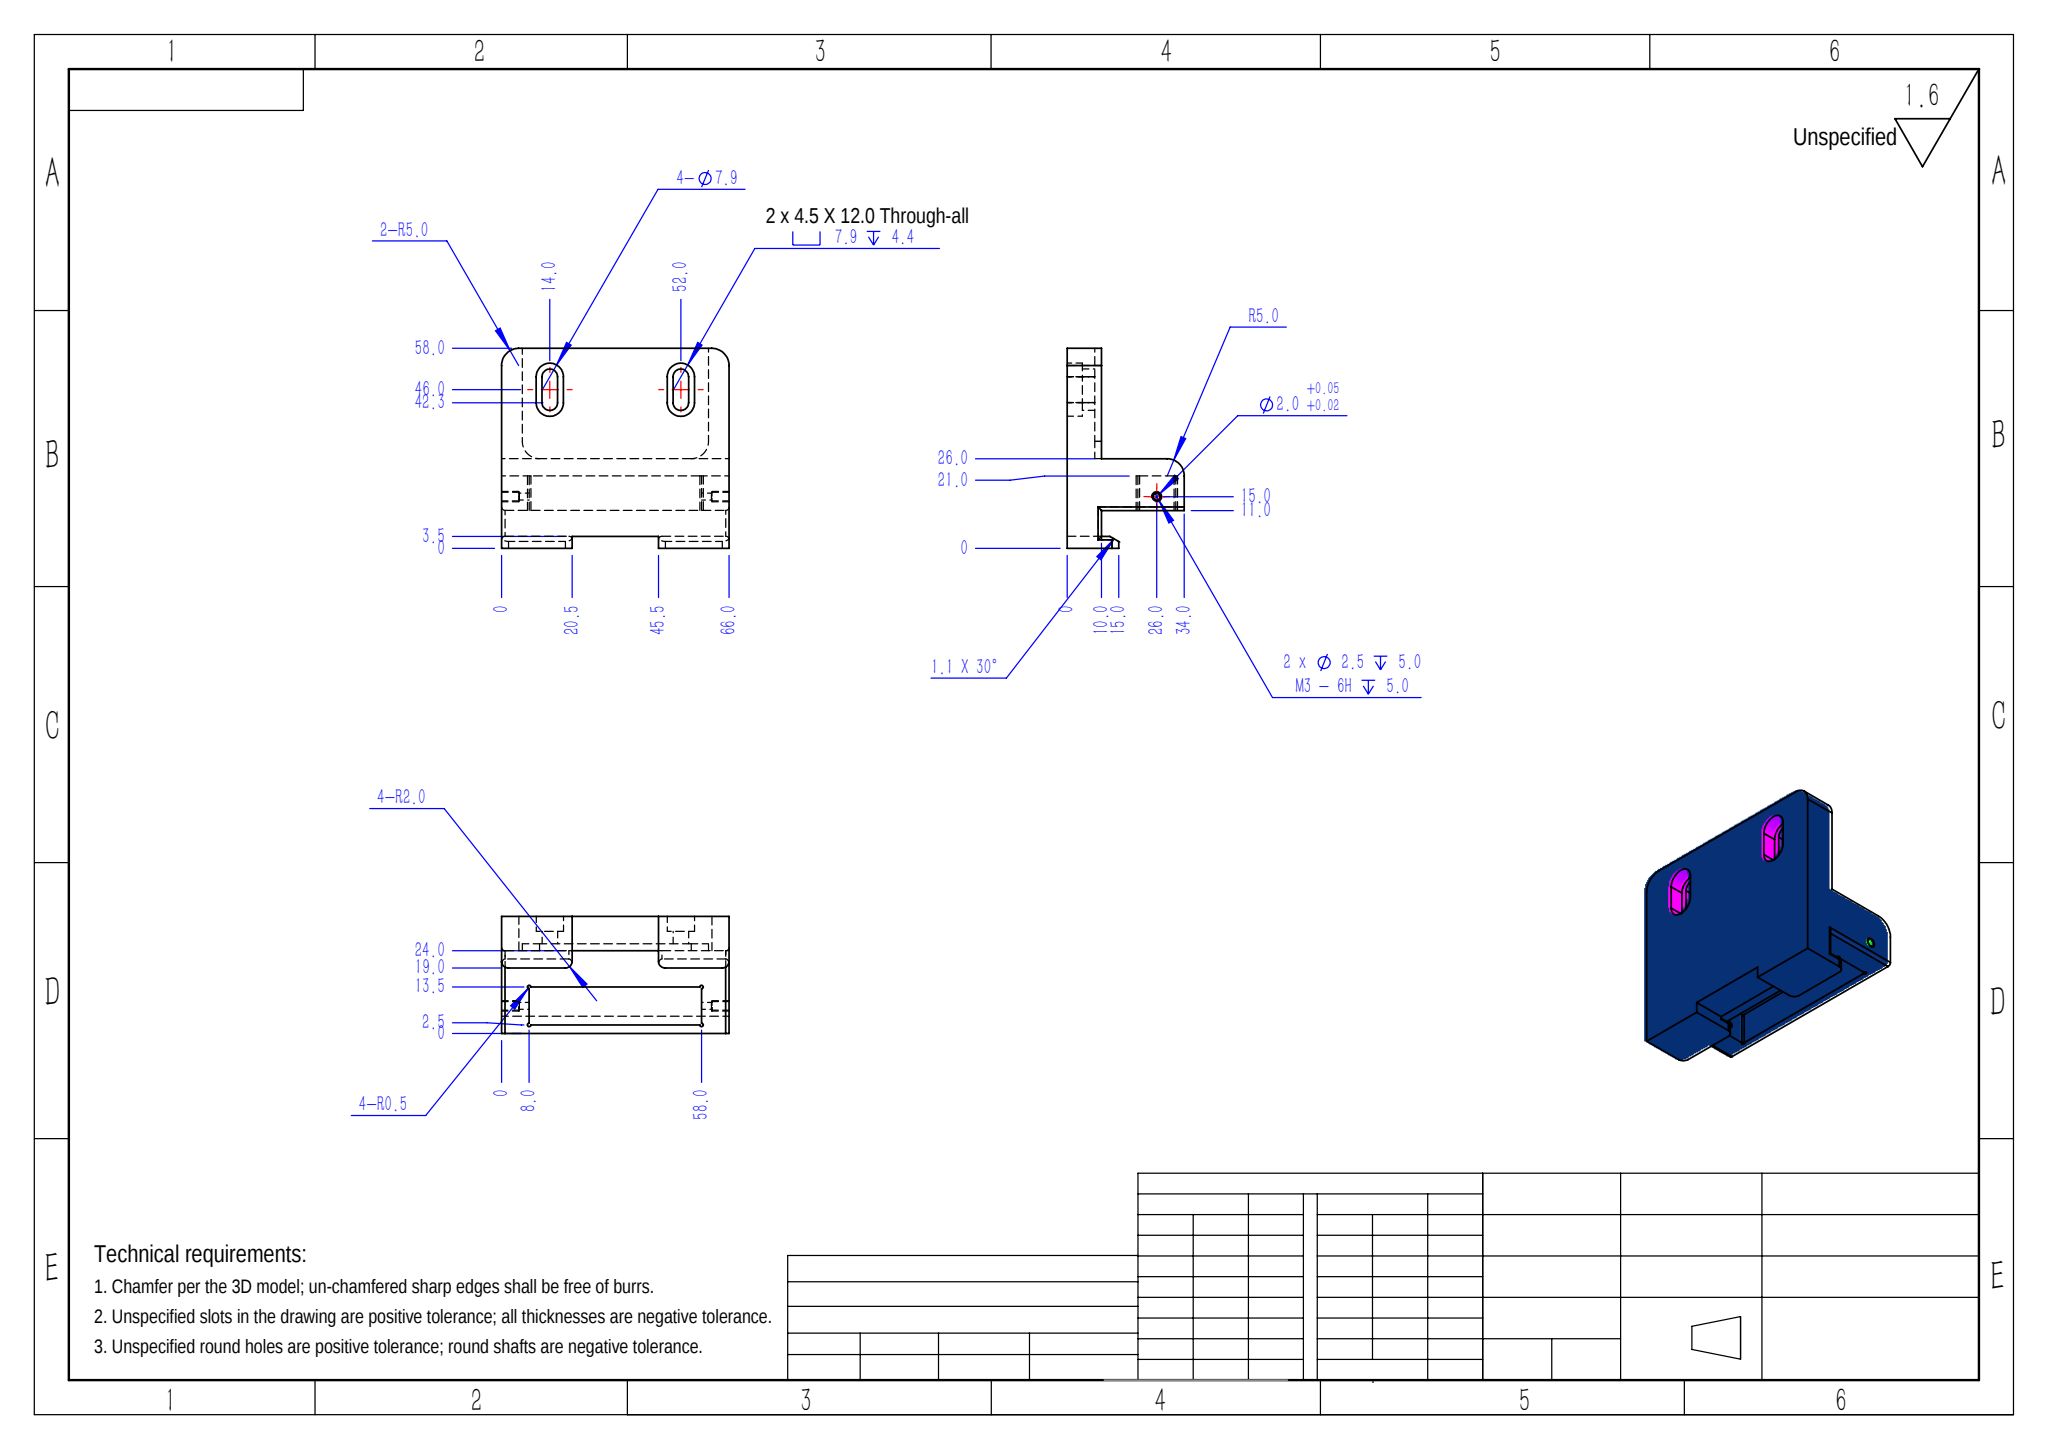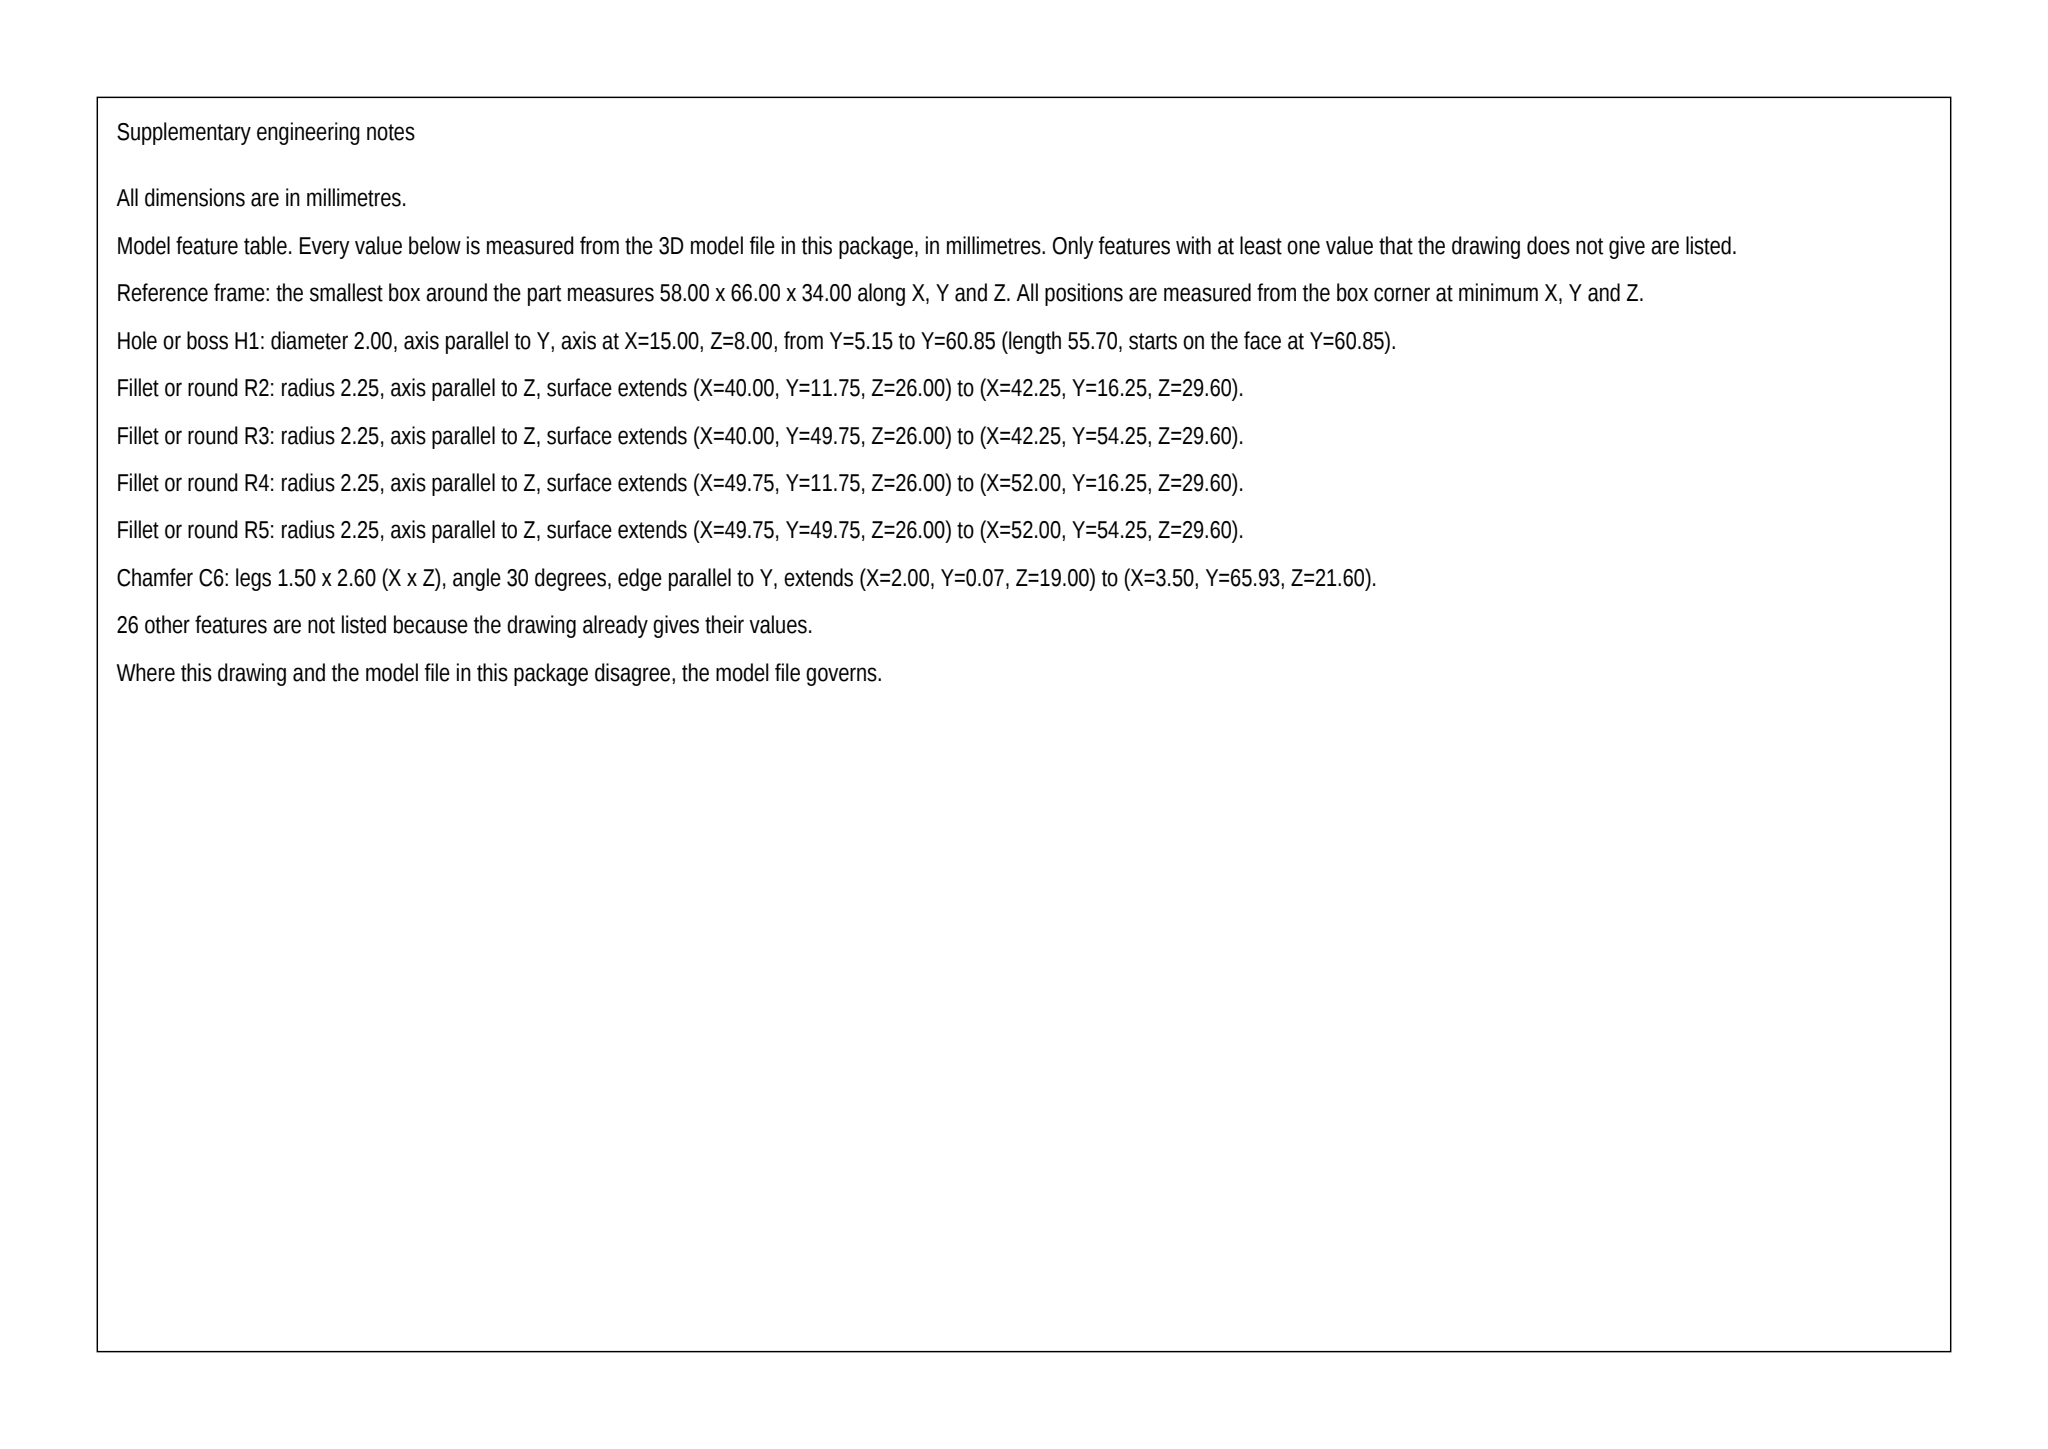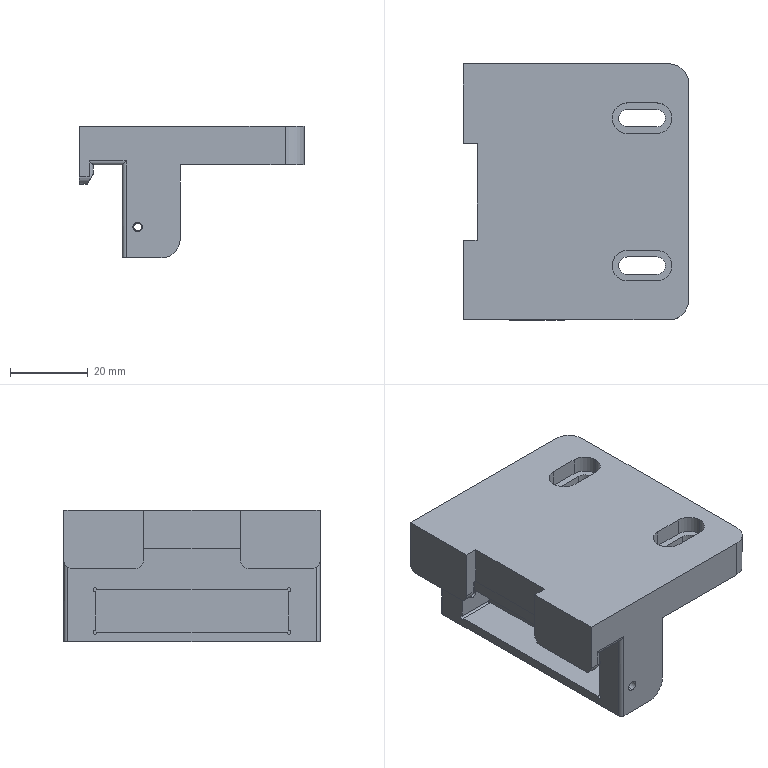Part | SolidWorks | mm | 1 solid | 86 faces | box 58 x 66 x 34 mm | volume 50981 mm3 | cylinder 43 | plane 39 | cone 4 | commonest cylinder face diameters 2 x12 7.9 x6 4.5 x6 1 x6 10 x5 2.5 x4 4 x4